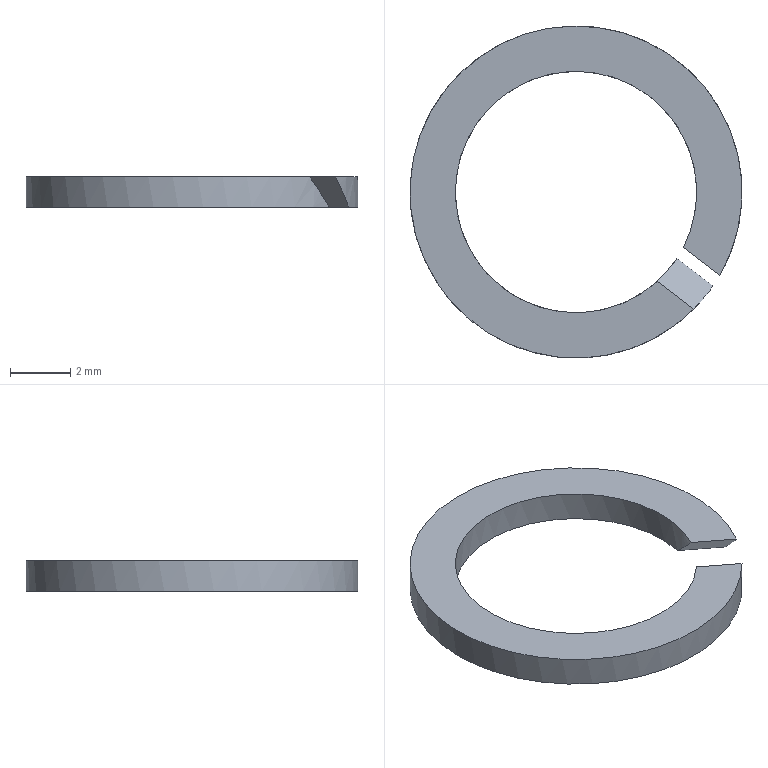Component | NX | SPRING_WASHER | 1 solid | 6 faces | box 11 x 11 x 1 mm | volume 43 mm3 | plane 4 | cylinder 2 | commonest cylinder face diameters 11 x1 8 x1
STEP:
#1=CARTESIAN_POINT('',(0.,0.,0.));
#2=DIRECTION('',(0.,0.,1.));
#3=DIRECTION('',(1.,0.,0.));
#4=AXIS2_PLACEMENT_3D('',#1,#2,#3);
#5=CARTESIAN_POINT('',(38.259,-39.131,-77.));
#6=VERTEX_POINT('',#5);
#7=CARTESIAN_POINT('',(37.398,-40.253,-77.));
#8=VERTEX_POINT('',#7);
#9=CARTESIAN_POINT('',(33.5,-36.373,-77.));
#10=DIRECTION('',(0.,0.,1.));
#11=DIRECTION('',(0.7936,-0.6084,0.));
#12=AXIS2_PLACEMENT_3D('',#9,#10,#11);
#13=CIRCLE('',#12,5.5);
#14=CARTESIAN_POINT('',(33.5,-36.373,-78.));
#15=DIRECTION('',(0.,0.,1.));
#16=DIRECTION('',(-0.7936,0.6084,0.));
#17=AXIS2_PLACEMENT_3D('',#14,#15,#16);
#18=CYLINDRICAL_SURFACE('',#17,5.5);
#19=CARTESIAN_POINT('',(-3.142,1.));
#20=DIRECTION('',(1.,0.));
#21=VECTOR('',#20,1.);
#22=LINE('',#19,#21);
#23=(GEOMETRIC_REPRESENTATION_CONTEXT(2)PARAMETRIC_REPRESENTATION_CONTEXT()REPRESENTATION_CONTEXT('',''));
#24=DEFINITIONAL_REPRESENTATION('',(#22),#23);
#25=PCURVE('',#18,#24);
#26=CARTESIAN_POINT('',(33.5,-36.373,-77.));
#27=DIRECTION('',(0.,0.,1.));
#28=DIRECTION('',(-0.7936,0.6084,0.));
#29=AXIS2_PLACEMENT_3D('',#26,#27,#28);
#30=PLANE('',#29);
#31=CARTESIAN_POINT('',(0.,0.));
#32=DIRECTION('',(-1.,0.));
#33=AXIS2_PLACEMENT_2D('',#31,#32);
#34=CIRCLE('',#33,5.5);
#35=(GEOMETRIC_REPRESENTATION_CONTEXT(2)PARAMETRIC_REPRESENTATION_CONTEXT()REPRESENTATION_CONTEXT('',''));
#36=DEFINITIONAL_REPRESENTATION('',(#34),#35);
#37=PCURVE('',#30,#36);
#38=SURFACE_CURVE('',#13,(#25,#37),.PCURVE_S1.);
#39=EDGE_CURVE('',#6,#8,#38,.T.);
#40=ORIENTED_EDGE('',*,*,#39,.F.);
#41=CARTESIAN_POINT('',(38.688,-38.2,-78.));
#42=VERTEX_POINT('',#41);
#43=CARTESIAN_POINT('',(33.5,-36.373,-76.293));
#44=DIRECTION('',(0.4302,0.5612,0.7071));
#45=DIRECTION('',(-0.4302,-0.5612,0.7071));
#46=AXIS2_PLACEMENT_3D('',#43,#44,#45);
#47=ELLIPSE('',#46,7.778,5.5);
#48=CARTESIAN_POINT('',(-3.013,1.));
#49=CARTESIAN_POINT('',(-2.826,0.));
#50=B_SPLINE_CURVE_WITH_KNOTS('',1,(#48,#49),.UNSPECIFIED.,.F.,.F.,(2,2),(1.7,1.886),.PIECEWISE_BEZIER_KNOTS.);
#51=(GEOMETRIC_REPRESENTATION_CONTEXT(2)PARAMETRIC_REPRESENTATION_CONTEXT()REPRESENTATION_CONTEXT('',''));
#52=DEFINITIONAL_REPRESENTATION('',(#50),#51);
#53=PCURVE('',#18,#52);
#54=CARTESIAN_POINT('',(42.152,-40.702,-78.122));
#55=DIRECTION('',(-0.4302,-0.5612,-0.7071));
#56=DIRECTION('',(0.4302,0.5612,-0.7071));
#57=AXIS2_PLACEMENT_3D('',#54,#55,#56);
#58=PLANE('',#57);
#59=CARTESIAN_POINT('',(-10.364,-9.5));
#60=CARTESIAN_POINT('',(-10.364,0.02628));
#61=CARTESIAN_POINT('',(1.303,-4.737));
#62=CARTESIAN_POINT('',(12.97,-9.5));
#63=CARTESIAN_POINT('',(1.303,-14.263));
#64=CARTESIAN_POINT('',(-10.364,-19.026));
#65=CARTESIAN_POINT('',(-10.364,-9.5));
#66=(BOUNDED_CURVE()B_SPLINE_CURVE(2,(#59,#60,#61,#62,#63,#64,#65),.UNSPECIFIED.,.T.,.F.)B_SPLINE_CURVE_WITH_KNOTS((1,2,2,2,2,1),(-2.094,0.,2.094,4.189,6.283,8.378),.UNSPECIFIED.)CURVE()GEOMETRIC_REPRESENTATION_ITEM()RATIONAL_B_SPLINE_CURVE((1.,0.5,1.,0.5,1.,0.5,1.))REPRESENTATION_ITEM(''));
#67=(GEOMETRIC_REPRESENTATION_CONTEXT(2)PARAMETRIC_REPRESENTATION_CONTEXT()REPRESENTATION_CONTEXT('',''));
#68=DEFINITIONAL_REPRESENTATION('',(#66),#67);
#69=PCURVE('',#58,#68);
#70=SURFACE_CURVE('',#47,(#53,#69),.PCURVE_S1.);
#71=EDGE_CURVE('',#6,#42,#70,.T.);
#72=ORIENTED_EDGE('',*,*,#71,.T.);
#73=CARTESIAN_POINT('',(38.037,-39.482,-78.));
#74=VERTEX_POINT('',#73);
#75=CARTESIAN_POINT('',(33.5,-36.373,-78.));
#76=DIRECTION('',(0.,0.,1.));
#77=DIRECTION('',(0.7936,-0.6084,0.));
#78=AXIS2_PLACEMENT_3D('',#75,#76,#77);
#79=CIRCLE('',#78,5.5);
#80=CARTESIAN_POINT('',(-3.142,0.));
#81=DIRECTION('',(1.,0.));
#82=VECTOR('',#81,1.);
#83=LINE('',#80,#82);
#84=(GEOMETRIC_REPRESENTATION_CONTEXT(2)PARAMETRIC_REPRESENTATION_CONTEXT()REPRESENTATION_CONTEXT('',''));
#85=DEFINITIONAL_REPRESENTATION('',(#83),#84);
#86=PCURVE('',#18,#85);
#87=CARTESIAN_POINT('',(33.5,-36.373,-78.));
#88=DIRECTION('',(0.,0.,1.));
#89=DIRECTION('',(-0.7936,0.6084,0.));
#90=AXIS2_PLACEMENT_3D('',#87,#88,#89);
#91=PLANE('',#90);
#92=CARTESIAN_POINT('',(0.,0.));
#93=DIRECTION('',(-1.,0.));
#94=AXIS2_PLACEMENT_2D('',#92,#93);
#95=CIRCLE('',#94,5.5);
#96=(GEOMETRIC_REPRESENTATION_CONTEXT(2)PARAMETRIC_REPRESENTATION_CONTEXT()REPRESENTATION_CONTEXT('',''));
#97=DEFINITIONAL_REPRESENTATION('',(#95),#96);
#98=PCURVE('',#91,#97);
#99=SURFACE_CURVE('',#79,(#86,#98),.PCURVE_S1.);
#100=EDGE_CURVE('',#42,#74,#99,.T.);
#101=ORIENTED_EDGE('',*,*,#100,.T.);
#102=CARTESIAN_POINT('',(33.5,-36.373,-77.707));
#103=DIRECTION('',(-0.4302,-0.5612,-0.7071));
#104=DIRECTION('',(-0.4302,-0.5612,0.7071));
#105=AXIS2_PLACEMENT_3D('',#102,#103,#104);
#106=ELLIPSE('',#105,7.778,5.5);
#107=CARTESIAN_POINT('',(3.195,0.));
#108=CARTESIAN_POINT('',(3.013,1.));
#109=B_SPLINE_CURVE_WITH_KNOTS('',1,(#107,#108),.UNSPECIFIED.,.F.,.F.,(2,2),(4.659,4.841),.PIECEWISE_BEZIER_KNOTS.);
#110=(GEOMETRIC_REPRESENTATION_CONTEXT(2)PARAMETRIC_REPRESENTATION_CONTEXT()REPRESENTATION_CONTEXT('',''));
#111=DEFINITIONAL_REPRESENTATION('',(#109),#110);
#112=PCURVE('',#18,#111);
#113=CARTESIAN_POINT('',(39.926,-43.605,-75.878));
#114=DIRECTION('',(0.4302,0.5612,0.7071));
#115=DIRECTION('',(-0.4302,-0.5612,0.7071));
#116=AXIS2_PLACEMENT_3D('',#113,#114,#115);
#117=PLANE('',#116);
#118=CARTESIAN_POINT('',(5.192,-9.5));
#119=CARTESIAN_POINT('',(5.192,-19.026));
#120=CARTESIAN_POINT('',(-6.475,-14.263));
#121=CARTESIAN_POINT('',(-18.143,-9.5));
#122=CARTESIAN_POINT('',(-6.475,-4.737));
#123=CARTESIAN_POINT('',(5.192,0.02628));
#124=CARTESIAN_POINT('',(5.192,-9.5));
#125=(BOUNDED_CURVE()B_SPLINE_CURVE(2,(#118,#119,#120,#121,#122,#123,#124),.UNSPECIFIED.,.T.,.F.)B_SPLINE_CURVE_WITH_KNOTS((1,2,2,2,2,1),(-2.094,0.,2.094,4.189,6.283,8.378),.UNSPECIFIED.)CURVE()GEOMETRIC_REPRESENTATION_ITEM()RATIONAL_B_SPLINE_CURVE((1.,0.5,1.,0.5,1.,0.5,1.))REPRESENTATION_ITEM(''));
#126=(GEOMETRIC_REPRESENTATION_CONTEXT(2)PARAMETRIC_REPRESENTATION_CONTEXT()REPRESENTATION_CONTEXT('',''));
#127=DEFINITIONAL_REPRESENTATION('',(#125),#126);
#128=PCURVE('',#117,#127);
#129=SURFACE_CURVE('',#106,(#112,#128),.PCURVE_S1.);
#130=EDGE_CURVE('',#74,#8,#129,.T.);
#131=ORIENTED_EDGE('',*,*,#130,.T.);
#132=EDGE_LOOP('',(#40,#72,#101,#131));
#133=FACE_BOUND('',#132,.T.);
#134=ADVANCED_FACE('',(#133),#18,.T.);
#135=CARTESIAN_POINT('',(37.409,-37.219,-78.));
#136=VERTEX_POINT('',#135);
#137=CARTESIAN_POINT('',(36.844,-38.568,-78.));
#138=VERTEX_POINT('',#137);
#139=CARTESIAN_POINT('',(33.5,-36.373,-78.));
#140=DIRECTION('',(0.,0.,1.));
#141=DIRECTION('',(0.7936,-0.6084,0.));
#142=AXIS2_PLACEMENT_3D('',#139,#140,#141);
#143=CIRCLE('',#142,4.);
#144=CARTESIAN_POINT('',(33.5,-36.373,-78.));
#145=DIRECTION('',(0.,0.,1.));
#146=DIRECTION('',(-0.7936,0.6084,0.));
#147=AXIS2_PLACEMENT_3D('',#144,#145,#146);
#148=CYLINDRICAL_SURFACE('',#147,4.);
#149=CARTESIAN_POINT('',(-3.142,0.));
#150=DIRECTION('',(1.,0.));
#151=VECTOR('',#150,1.);
#152=LINE('',#149,#151);
#153=(GEOMETRIC_REPRESENTATION_CONTEXT(2)PARAMETRIC_REPRESENTATION_CONTEXT()REPRESENTATION_CONTEXT('',''));
#154=DEFINITIONAL_REPRESENTATION('',(#152),#153);
#155=PCURVE('',#148,#154);
#156=CARTESIAN_POINT('',(0.,0.));
#157=DIRECTION('',(-1.,0.));
#158=AXIS2_PLACEMENT_2D('',#156,#157);
#159=CIRCLE('',#158,4.);
#160=(GEOMETRIC_REPRESENTATION_CONTEXT(2)PARAMETRIC_REPRESENTATION_CONTEXT()REPRESENTATION_CONTEXT('',''));
#161=DEFINITIONAL_REPRESENTATION('',(#159),#160);
#162=PCURVE('',#91,#161);
#163=SURFACE_CURVE('',#143,(#155,#162),.PCURVE_S1.);
#164=EDGE_CURVE('',#136,#138,#163,.T.);
#165=ORIENTED_EDGE('',*,*,#164,.T.);
#166=CARTESIAN_POINT('',(36.194,-39.33,-77.));
#167=VERTEX_POINT('',#166);
#168=CARTESIAN_POINT('',(33.5,-36.373,-77.707));
#169=DIRECTION('',(-0.4302,-0.5612,-0.7071));
#170=DIRECTION('',(-0.4302,-0.5612,0.7071));
#171=AXIS2_PLACEMENT_3D('',#168,#169,#170);
#172=ELLIPSE('',#171,5.657,4.);
#173=CARTESIAN_POINT('',(3.215,0.));
#174=CARTESIAN_POINT('',(2.964,1.));
#175=B_SPLINE_CURVE_WITH_KNOTS('',1,(#173,#174),.UNSPECIFIED.,.F.,.F.,(2,2),(4.639,4.89),.PIECEWISE_BEZIER_KNOTS.);
#176=(GEOMETRIC_REPRESENTATION_CONTEXT(2)PARAMETRIC_REPRESENTATION_CONTEXT()REPRESENTATION_CONTEXT('',''));
#177=DEFINITIONAL_REPRESENTATION('',(#175),#176);
#178=PCURVE('',#148,#177);
#179=CARTESIAN_POINT('',(3.071,-9.5));
#180=CARTESIAN_POINT('',(3.071,-16.428));
#181=CARTESIAN_POINT('',(-5.415,-12.964));
#182=CARTESIAN_POINT('',(-13.9,-9.5));
#183=CARTESIAN_POINT('',(-5.415,-6.036));
#184=CARTESIAN_POINT('',(3.071,-2.572));
#185=CARTESIAN_POINT('',(3.071,-9.5));
#186=(BOUNDED_CURVE()B_SPLINE_CURVE(2,(#179,#180,#181,#182,#183,#184,#185),.UNSPECIFIED.,.T.,.F.)B_SPLINE_CURVE_WITH_KNOTS((1,2,2,2,2,1),(-2.094,0.,2.094,4.189,6.283,8.378),.UNSPECIFIED.)CURVE()GEOMETRIC_REPRESENTATION_ITEM()RATIONAL_B_SPLINE_CURVE((1.,0.5,1.,0.5,1.,0.5,1.))REPRESENTATION_ITEM(''));
#187=(GEOMETRIC_REPRESENTATION_CONTEXT(2)PARAMETRIC_REPRESENTATION_CONTEXT()REPRESENTATION_CONTEXT('',''));
#188=DEFINITIONAL_REPRESENTATION('',(#186),#187);
#189=PCURVE('',#117,#188);
#190=SURFACE_CURVE('',#172,(#178,#189),.PCURVE_S1.);
#191=EDGE_CURVE('',#138,#167,#190,.T.);
#192=ORIENTED_EDGE('',*,*,#191,.T.);
#193=CARTESIAN_POINT('',(37.055,-38.207,-77.));
#194=VERTEX_POINT('',#193);
#195=CARTESIAN_POINT('',(33.5,-36.373,-77.));
#196=DIRECTION('',(0.,0.,1.));
#197=DIRECTION('',(0.7936,-0.6084,0.));
#198=AXIS2_PLACEMENT_3D('',#195,#196,#197);
#199=CIRCLE('',#198,4.);
#200=CARTESIAN_POINT('',(-3.142,1.));
#201=DIRECTION('',(1.,0.));
#202=VECTOR('',#201,1.);
#203=LINE('',#200,#202);
#204=(GEOMETRIC_REPRESENTATION_CONTEXT(2)PARAMETRIC_REPRESENTATION_CONTEXT()REPRESENTATION_CONTEXT('',''));
#205=DEFINITIONAL_REPRESENTATION('',(#203),#204);
#206=PCURVE('',#148,#205);
#207=CARTESIAN_POINT('',(0.,0.));
#208=DIRECTION('',(-1.,0.));
#209=AXIS2_PLACEMENT_2D('',#207,#208);
#210=CIRCLE('',#209,4.);
#211=(GEOMETRIC_REPRESENTATION_CONTEXT(2)PARAMETRIC_REPRESENTATION_CONTEXT()REPRESENTATION_CONTEXT('',''));
#212=DEFINITIONAL_REPRESENTATION('',(#210),#211);
#213=PCURVE('',#30,#212);
#214=SURFACE_CURVE('',#199,(#206,#213),.PCURVE_S1.);
#215=EDGE_CURVE('',#194,#167,#214,.T.);
#216=ORIENTED_EDGE('',*,*,#215,.F.);
#217=CARTESIAN_POINT('',(33.5,-36.373,-76.293));
#218=DIRECTION('',(0.4302,0.5612,0.7071));
#219=DIRECTION('',(-0.4302,-0.5612,0.7071));
#220=AXIS2_PLACEMENT_3D('',#217,#218,#219);
#221=ELLIPSE('',#220,5.657,4.);
#222=CARTESIAN_POINT('',(-2.964,1.));
#223=CARTESIAN_POINT('',(-2.701,0.));
#224=B_SPLINE_CURVE_WITH_KNOTS('',1,(#222,#223),.UNSPECIFIED.,.F.,.F.,(2,2),(1.749,2.012),.PIECEWISE_BEZIER_KNOTS.);
#225=(GEOMETRIC_REPRESENTATION_CONTEXT(2)PARAMETRIC_REPRESENTATION_CONTEXT()REPRESENTATION_CONTEXT('',''));
#226=DEFINITIONAL_REPRESENTATION('',(#224),#225);
#227=PCURVE('',#148,#226);
#228=CARTESIAN_POINT('',(-8.243,-9.5));
#229=CARTESIAN_POINT('',(-8.243,-2.572));
#230=CARTESIAN_POINT('',(0.2422,-6.036));
#231=CARTESIAN_POINT('',(8.727,-9.5));
#232=CARTESIAN_POINT('',(0.2422,-12.964));
#233=CARTESIAN_POINT('',(-8.243,-16.428));
#234=CARTESIAN_POINT('',(-8.243,-9.5));
#235=(BOUNDED_CURVE()B_SPLINE_CURVE(2,(#228,#229,#230,#231,#232,#233,#234),.UNSPECIFIED.,.T.,.F.)B_SPLINE_CURVE_WITH_KNOTS((1,2,2,2,2,1),(-2.094,0.,2.094,4.189,6.283,8.378),.UNSPECIFIED.)CURVE()GEOMETRIC_REPRESENTATION_ITEM()RATIONAL_B_SPLINE_CURVE((1.,0.5,1.,0.5,1.,0.5,1.))REPRESENTATION_ITEM(''));
#236=(GEOMETRIC_REPRESENTATION_CONTEXT(2)PARAMETRIC_REPRESENTATION_CONTEXT()REPRESENTATION_CONTEXT('',''));
#237=DEFINITIONAL_REPRESENTATION('',(#235),#236);
#238=PCURVE('',#58,#237);
#239=SURFACE_CURVE('',#221,(#227,#238),.PCURVE_S1.);
#240=EDGE_CURVE('',#194,#136,#239,.T.);
#241=ORIENTED_EDGE('',*,*,#240,.T.);
#242=EDGE_LOOP('',(#165,#192,#216,#241));
#243=FACE_BOUND('',#242,.F.);
#244=ADVANCED_FACE('',(#243),#148,.F.);
#245=CARTESIAN_POINT('',(34.539,-35.018,-78.));
#246=DIRECTION('',(0.7936,-0.6084,0.));
#247=VECTOR('',#246,1.);
#248=LINE('',#245,#247);
#249=CARTESIAN_POINT('',(0.,-1.707));
#250=DIRECTION('',(-1.,0.));
#251=VECTOR('',#250,1.);
#252=LINE('',#249,#251);
#253=(GEOMETRIC_REPRESENTATION_CONTEXT(2)PARAMETRIC_REPRESENTATION_CONTEXT()REPRESENTATION_CONTEXT('',''));
#254=DEFINITIONAL_REPRESENTATION('',(#252),#253);
#255=PCURVE('',#91,#254);
#256=CARTESIAN_POINT('',(-0.172,-9.5));
#257=DIRECTION('',(0.,1.));
#258=VECTOR('',#257,1.);
#259=LINE('',#256,#258);
#260=(GEOMETRIC_REPRESENTATION_CONTEXT(2)PARAMETRIC_REPRESENTATION_CONTEXT()REPRESENTATION_CONTEXT('',''));
#261=DEFINITIONAL_REPRESENTATION('',(#259),#260);
#262=PCURVE('',#58,#261);
#263=SURFACE_CURVE('',#248,(#255,#262),.PCURVE_S1.);
#264=EDGE_CURVE('',#136,#42,#263,.T.);
#265=ORIENTED_EDGE('',*,*,#264,.F.);
#266=ORIENTED_EDGE('',*,*,#164,.T.);
#267=CARTESIAN_POINT('',(33.678,-36.141,-78.));
#268=DIRECTION('',(-0.7936,0.6084,0.));
#269=VECTOR('',#268,1.);
#270=LINE('',#267,#269);
#271=CARTESIAN_POINT('',(0.,-0.2929));
#272=DIRECTION('',(1.,0.));
#273=VECTOR('',#272,1.);
#274=LINE('',#271,#273);
#275=(GEOMETRIC_REPRESENTATION_CONTEXT(2)PARAMETRIC_REPRESENTATION_CONTEXT()REPRESENTATION_CONTEXT('',''));
#276=DEFINITIONAL_REPRESENTATION('',(#274),#275);
#277=PCURVE('',#91,#276);
#278=CARTESIAN_POINT('',(-3.,-9.5));
#279=DIRECTION('',(0.,-1.));
#280=VECTOR('',#279,1.);
#281=LINE('',#278,#280);
#282=(GEOMETRIC_REPRESENTATION_CONTEXT(2)PARAMETRIC_REPRESENTATION_CONTEXT()REPRESENTATION_CONTEXT('',''));
#283=DEFINITIONAL_REPRESENTATION('',(#281),#282);
#284=PCURVE('',#117,#283);
#285=SURFACE_CURVE('',#270,(#277,#284),.PCURVE_S1.);
#286=EDGE_CURVE('',#74,#138,#285,.T.);
#287=ORIENTED_EDGE('',*,*,#286,.F.);
#288=ORIENTED_EDGE('',*,*,#100,.F.);
#289=EDGE_LOOP('',(#265,#266,#287,#288));
#290=FACE_BOUND('',#289,.T.);
#291=ADVANCED_FACE('',(#290),#91,.F.);
#292=ORIENTED_EDGE('',*,*,#215,.F.);
#293=CARTESIAN_POINT('',(33.93,-35.812,-77.));
#294=DIRECTION('',(0.7936,-0.6084,0.));
#295=VECTOR('',#294,1.);
#296=LINE('',#293,#295);
#297=CARTESIAN_POINT('',(-0.,-0.7071));
#298=DIRECTION('',(-1.,0.));
#299=VECTOR('',#298,1.);
#300=LINE('',#297,#299);
#301=(GEOMETRIC_REPRESENTATION_CONTEXT(2)PARAMETRIC_REPRESENTATION_CONTEXT()REPRESENTATION_CONTEXT('',''));
#302=DEFINITIONAL_REPRESENTATION('',(#300),#301);
#303=PCURVE('',#30,#302);
#304=CARTESIAN_POINT('',(-1.586,-9.5));
#305=DIRECTION('',(0.,1.));
#306=VECTOR('',#305,1.);
#307=LINE('',#304,#306);
#308=(GEOMETRIC_REPRESENTATION_CONTEXT(2)PARAMETRIC_REPRESENTATION_CONTEXT()REPRESENTATION_CONTEXT('',''));
#309=DEFINITIONAL_REPRESENTATION('',(#307),#308);
#310=PCURVE('',#58,#309);
#311=SURFACE_CURVE('',#296,(#303,#310),.PCURVE_S1.);
#312=EDGE_CURVE('',#194,#6,#311,.T.);
#313=ORIENTED_EDGE('',*,*,#312,.T.);
#314=ORIENTED_EDGE('',*,*,#39,.T.);
#315=CARTESIAN_POINT('',(33.07,-36.934,-77.));
#316=DIRECTION('',(-0.7936,0.6084,0.));
#317=VECTOR('',#316,1.);
#318=LINE('',#315,#317);
#319=CARTESIAN_POINT('',(0.,0.7071));
#320=DIRECTION('',(1.,0.));
#321=VECTOR('',#320,1.);
#322=LINE('',#319,#321);
#323=(GEOMETRIC_REPRESENTATION_CONTEXT(2)PARAMETRIC_REPRESENTATION_CONTEXT()REPRESENTATION_CONTEXT('',''));
#324=DEFINITIONAL_REPRESENTATION('',(#322),#323);
#325=PCURVE('',#30,#324);
#326=CARTESIAN_POINT('',(-1.586,-9.5));
#327=DIRECTION('',(0.,-1.));
#328=VECTOR('',#327,1.);
#329=LINE('',#326,#328);
#330=(GEOMETRIC_REPRESENTATION_CONTEXT(2)PARAMETRIC_REPRESENTATION_CONTEXT()REPRESENTATION_CONTEXT('',''));
#331=DEFINITIONAL_REPRESENTATION('',(#329),#330);
#332=PCURVE('',#117,#331);
#333=SURFACE_CURVE('',#318,(#325,#332),.PCURVE_S1.);
#334=EDGE_CURVE('',#8,#167,#333,.T.);
#335=ORIENTED_EDGE('',*,*,#334,.T.);
#336=EDGE_LOOP('',(#292,#313,#314,#335));
#337=FACE_BOUND('',#336,.T.);
#338=ADVANCED_FACE('',(#337),#30,.T.);
#339=ORIENTED_EDGE('',*,*,#286,.T.);
#340=ORIENTED_EDGE('',*,*,#191,.T.);
#341=ORIENTED_EDGE('',*,*,#334,.F.);
#342=ORIENTED_EDGE('',*,*,#130,.F.);
#343=EDGE_LOOP('',(#339,#340,#341,#342));
#344=FACE_BOUND('',#343,.T.);
#345=ADVANCED_FACE('',(#344),#117,.T.);
#346=ORIENTED_EDGE('',*,*,#264,.T.);
#347=ORIENTED_EDGE('',*,*,#71,.F.);
#348=ORIENTED_EDGE('',*,*,#312,.F.);
#349=ORIENTED_EDGE('',*,*,#240,.T.);
#350=EDGE_LOOP('',(#346,#347,#348,#349));
#351=FACE_BOUND('',#350,.T.);
#352=ADVANCED_FACE('',(#351),#58,.T.);
#353=CLOSED_SHELL('',(#134,#244,#291,#338,#345,#352));
#354=MANIFOLD_SOLID_BREP('',#353);
#355=(LENGTH_UNIT()NAMED_UNIT(*)SI_UNIT(.MILLI.,.METRE.));
#356=UNCERTAINTY_MEASURE_WITH_UNIT(LENGTH_MEASURE(0.005),#355,'','');
#357=(NAMED_UNIT(*)PLANE_ANGLE_UNIT()SI_UNIT($,.RADIAN.));
#358=(NAMED_UNIT(*)SI_UNIT($,.STERADIAN.)SOLID_ANGLE_UNIT());
#359=(GEOMETRIC_REPRESENTATION_CONTEXT(3)GLOBAL_UNCERTAINTY_ASSIGNED_CONTEXT((#356))GLOBAL_UNIT_ASSIGNED_CONTEXT((#355,#357,#358))REPRESENTATION_CONTEXT('',''));
#360=ADVANCED_BREP_SHAPE_REPRESENTATION('',(#4,#354),#359);